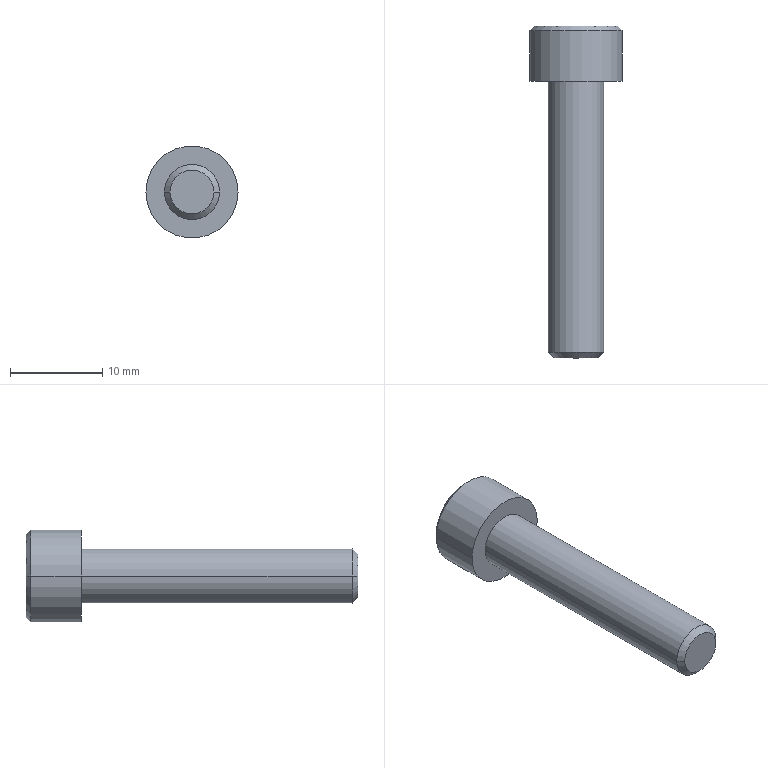Component | SolidWorks | TAD01-M6-L30Screw-2 | 1 solid | 25 faces | box 10 x 36 x 10 mm | volume 1238 mm3 | plane 15 | cone 6 | cylinder 4 | commonest cylinder face diameters 6 x2 10 x2
STEP:
#1=COLOUR_RGB('',0.7922,0.8196,0.9333);
#2=FILL_AREA_STYLE_COLOUR('',#1);
#3=FILL_AREA_STYLE('',(#2));
#4=SURFACE_STYLE_FILL_AREA(#3);
#5=SURFACE_SIDE_STYLE('',(#4));
#6=SURFACE_STYLE_USAGE(.BOTH.,#5);
#7=PRESENTATION_STYLE_ASSIGNMENT((#6));
#8=CARTESIAN_POINT('',(-0.1442,1.796,7.539));
#9=VERTEX_POINT('',#8);
#10=CARTESIAN_POINT('',(-0.3805,1.796,7.539));
#11=VERTEX_POINT('',#10);
#12=CARTESIAN_POINT('',(-0.2623,1.796,7.539));
#13=DIRECTION('',(0.,1.,0.));
#14=DIRECTION('',(1.,0.,0.));
#15=AXIS2_PLACEMENT_3D('',#12,#13,#14);
#16=CIRCLE('',#15,0.1181);
#17=EDGE_CURVE('',#9,#11,#16,.T.);
#18=ORIENTED_EDGE('',*,*,#17,.T.);
#19=CARTESIAN_POINT('',(-0.3805,2.953,7.539));
#20=VERTEX_POINT('',#19);
#21=CARTESIAN_POINT('',(-0.3805,1.771,7.539));
#22=DIRECTION('',(0.,1.,0.));
#23=VECTOR('',#22,39.37);
#24=LINE('',#21,#23);
#25=EDGE_CURVE('',#11,#20,#24,.T.);
#26=ORIENTED_EDGE('',*,*,#25,.T.);
#27=CARTESIAN_POINT('',(-0.1442,2.953,7.539));
#28=VERTEX_POINT('',#27);
#29=CARTESIAN_POINT('',(-0.2623,2.953,7.539));
#30=DIRECTION('',(0.,-1.,0.));
#31=DIRECTION('',(1.,0.,0.));
#32=AXIS2_PLACEMENT_3D('',#29,#30,#31);
#33=CIRCLE('',#32,0.1181);
#34=EDGE_CURVE('',#20,#28,#33,.T.);
#35=ORIENTED_EDGE('',*,*,#34,.T.);
#36=CARTESIAN_POINT('',(-0.1442,1.771,7.539));
#37=DIRECTION('',(0.,1.,0.));
#38=VECTOR('',#37,39.37);
#39=LINE('',#36,#38);
#40=EDGE_CURVE('',#9,#28,#39,.T.);
#41=ORIENTED_EDGE('',*,*,#40,.F.);
#42=EDGE_LOOP('',(#18,#26,#35,#41));
#43=FACE_OUTER_BOUND('',#42,.T.);
#44=CARTESIAN_POINT('',(-0.2623,1.771,7.539));
#45=DIRECTION('',(0.,1.,0.));
#46=DIRECTION('',(1.,0.,0.));
#47=AXIS2_PLACEMENT_3D('',#44,#45,#46);
#48=CYLINDRICAL_SURFACE('',#47,0.1181);
#49=ADVANCED_FACE('',(#43),#48,.T.);
#50=CARTESIAN_POINT('',(-0.1684,1.771,7.539));
#51=VERTEX_POINT('',#50);
#52=CARTESIAN_POINT('',(-0.3563,1.771,7.539));
#53=VERTEX_POINT('',#52);
#54=CARTESIAN_POINT('',(-0.2623,1.771,7.539));
#55=DIRECTION('',(0.,1.,0.));
#56=DIRECTION('',(1.,0.,0.));
#57=AXIS2_PLACEMENT_3D('',#54,#55,#56);
#58=CIRCLE('',#57,0.09396);
#59=EDGE_CURVE('',#51,#53,#58,.T.);
#60=ORIENTED_EDGE('',*,*,#59,.T.);
#61=CARTESIAN_POINT('',(-0.3805,1.796,7.539));
#62=DIRECTION('',(-0.7071,0.7071,-0.));
#63=VECTOR('',#62,39.37);
#64=LINE('',#61,#63);
#65=EDGE_CURVE('',#53,#11,#64,.T.);
#66=ORIENTED_EDGE('',*,*,#65,.T.);
#67=ORIENTED_EDGE('',*,*,#17,.F.);
#68=CARTESIAN_POINT('',(-0.1442,1.796,7.539));
#69=DIRECTION('',(0.7071,0.7071,0.));
#70=VECTOR('',#69,39.37);
#71=LINE('',#68,#70);
#72=EDGE_CURVE('',#51,#9,#71,.T.);
#73=ORIENTED_EDGE('',*,*,#72,.F.);
#74=EDGE_LOOP('',(#60,#66,#67,#73));
#75=FACE_OUTER_BOUND('',#74,.T.);
#76=CARTESIAN_POINT('',(-0.2623,1.796,7.539));
#77=DIRECTION('',(0.,1.,0.));
#78=DIRECTION('',(1.,0.,0.));
#79=AXIS2_PLACEMENT_3D('',#76,#77,#78);
#80=CONICAL_SURFACE('',#79,0.1181,0.7854);
#81=ADVANCED_FACE('',(#75),#80,.T.);
#82=CARTESIAN_POINT('',(-0.06549,2.953,7.539));
#83=VERTEX_POINT('',#82);
#84=CARTESIAN_POINT('',(-0.4592,2.953,7.539));
#85=VERTEX_POINT('',#84);
#86=CARTESIAN_POINT('',(-0.2623,2.953,7.539));
#87=DIRECTION('',(0.,1.,0.));
#88=DIRECTION('',(1.,0.,0.));
#89=AXIS2_PLACEMENT_3D('',#86,#87,#88);
#90=CIRCLE('',#89,0.1969);
#91=EDGE_CURVE('',#83,#85,#90,.T.);
#92=ORIENTED_EDGE('',*,*,#91,.T.);
#93=CARTESIAN_POINT('',(-0.4592,3.169,7.539));
#94=VERTEX_POINT('',#93);
#95=CARTESIAN_POINT('',(-0.4592,2.953,7.539));
#96=DIRECTION('',(0.,1.,0.));
#97=VECTOR('',#96,39.37);
#98=LINE('',#95,#97);
#99=EDGE_CURVE('',#85,#94,#98,.T.);
#100=ORIENTED_EDGE('',*,*,#99,.T.);
#101=CARTESIAN_POINT('',(-0.06549,3.169,7.539));
#102=VERTEX_POINT('',#101);
#103=CARTESIAN_POINT('',(-0.2623,3.169,7.539));
#104=DIRECTION('',(0.,-1.,0.));
#105=DIRECTION('',(1.,0.,0.));
#106=AXIS2_PLACEMENT_3D('',#103,#104,#105);
#107=CIRCLE('',#106,0.1969);
#108=EDGE_CURVE('',#94,#102,#107,.T.);
#109=ORIENTED_EDGE('',*,*,#108,.T.);
#110=CARTESIAN_POINT('',(-0.06549,2.953,7.539));
#111=DIRECTION('',(0.,1.,0.));
#112=VECTOR('',#111,39.37);
#113=LINE('',#110,#112);
#114=EDGE_CURVE('',#83,#102,#113,.T.);
#115=ORIENTED_EDGE('',*,*,#114,.F.);
#116=EDGE_LOOP('',(#92,#100,#109,#115));
#117=FACE_OUTER_BOUND('',#116,.T.);
#118=CARTESIAN_POINT('',(-0.2623,2.953,7.539));
#119=DIRECTION('',(0.,1.,0.));
#120=DIRECTION('',(1.,0.,0.));
#121=AXIS2_PLACEMENT_3D('',#118,#119,#120);
#122=CYLINDRICAL_SURFACE('',#121,0.1969);
#123=ADVANCED_FACE('',(#117),#122,.T.);
#124=CARTESIAN_POINT('',(-0.4395,3.189,7.539));
#125=VERTEX_POINT('',#124);
#126=CARTESIAN_POINT('',(-0.08518,3.189,7.539));
#127=VERTEX_POINT('',#126);
#128=CARTESIAN_POINT('',(-0.2623,3.189,7.539));
#129=DIRECTION('',(0.,-1.,0.));
#130=DIRECTION('',(-1.,0.,0.));
#131=AXIS2_PLACEMENT_3D('',#128,#129,#130);
#132=CIRCLE('',#131,0.1772);
#133=EDGE_CURVE('',#125,#127,#132,.T.);
#134=ORIENTED_EDGE('',*,*,#133,.T.);
#135=CARTESIAN_POINT('',(-0.06549,3.169,7.539));
#136=DIRECTION('',(0.7071,-0.7071,-0.));
#137=VECTOR('',#136,39.37);
#138=LINE('',#135,#137);
#139=EDGE_CURVE('',#127,#102,#138,.T.);
#140=ORIENTED_EDGE('',*,*,#139,.T.);
#141=ORIENTED_EDGE('',*,*,#108,.F.);
#142=CARTESIAN_POINT('',(-0.4592,3.169,7.539));
#143=DIRECTION('',(-0.7071,-0.7071,0.));
#144=VECTOR('',#143,39.37);
#145=LINE('',#142,#144);
#146=EDGE_CURVE('',#125,#94,#145,.T.);
#147=ORIENTED_EDGE('',*,*,#146,.F.);
#148=EDGE_LOOP('',(#134,#140,#141,#147));
#149=FACE_OUTER_BOUND('',#148,.T.);
#150=CARTESIAN_POINT('',(-0.2623,3.169,7.539));
#151=DIRECTION('',(0.,-1.,0.));
#152=DIRECTION('',(-1.,0.,0.));
#153=AXIS2_PLACEMENT_3D('',#150,#151,#152);
#154=CONICAL_SURFACE('',#153,0.1969,0.7854);
#155=ADVANCED_FACE('',(#149),#154,.T.);
#156=CARTESIAN_POINT('',(-0.2623,3.014,7.539));
#157=VERTEX_POINT('',#156);
#158=CARTESIAN_POINT('',(-0.2623,3.071,7.638));
#159=VERTEX_POINT('',#158);
#160=CARTESIAN_POINT('',(-0.2623,3.071,7.638));
#161=DIRECTION('',(0.,0.5,0.866));
#162=VECTOR('',#161,39.37);
#163=LINE('',#160,#162);
#164=EDGE_CURVE('',#157,#159,#163,.T.);
#165=ORIENTED_EDGE('',*,*,#164,.F.);
#166=CARTESIAN_POINT('',(-0.2623,3.071,7.441));
#167=VERTEX_POINT('',#166);
#168=CARTESIAN_POINT('',(-0.2623,3.071,7.441));
#169=DIRECTION('',(0.,0.5,-0.866));
#170=VECTOR('',#169,39.37);
#171=LINE('',#168,#170);
#172=EDGE_CURVE('',#157,#167,#171,.T.);
#173=ORIENTED_EDGE('',*,*,#172,.T.);
#174=CARTESIAN_POINT('',(-0.3116,3.071,7.454));
#175=VERTEX_POINT('',#174);
#176=CARTESIAN_POINT('',(-0.2623,3.071,7.539));
#177=DIRECTION('',(-0.,-1.,-0.));
#178=DIRECTION('',(0.,0.,1.));
#179=AXIS2_PLACEMENT_3D('',#176,#177,#178);
#180=CIRCLE('',#179,0.09843);
#181=EDGE_CURVE('',#175,#167,#180,.T.);
#182=ORIENTED_EDGE('',*,*,#181,.F.);
#183=CARTESIAN_POINT('',(-0.3608,3.071,7.539));
#184=VERTEX_POINT('',#183);
#185=CARTESIAN_POINT('',(-0.2623,3.071,7.539));
#186=DIRECTION('',(-0.,-1.,-0.));
#187=DIRECTION('',(-0.,0.,1.));
#188=AXIS2_PLACEMENT_3D('',#185,#186,#187);
#189=CIRCLE('',#188,0.09843);
#190=EDGE_CURVE('',#184,#175,#189,.T.);
#191=ORIENTED_EDGE('',*,*,#190,.F.);
#192=CARTESIAN_POINT('',(-0.3116,3.071,7.625));
#193=VERTEX_POINT('',#192);
#194=CARTESIAN_POINT('',(-0.2623,3.071,7.539));
#195=DIRECTION('',(-0.,-1.,-0.));
#196=DIRECTION('',(0.,0.,1.));
#197=AXIS2_PLACEMENT_3D('',#194,#195,#196);
#198=CIRCLE('',#197,0.09843);
#199=EDGE_CURVE('',#193,#184,#198,.T.);
#200=ORIENTED_EDGE('',*,*,#199,.F.);
#201=CARTESIAN_POINT('',(-0.2623,3.071,7.539));
#202=DIRECTION('',(-0.,-1.,-0.));
#203=DIRECTION('',(0.,0.,1.));
#204=AXIS2_PLACEMENT_3D('',#201,#202,#203);
#205=CIRCLE('',#204,0.09843);
#206=EDGE_CURVE('',#159,#193,#205,.T.);
#207=ORIENTED_EDGE('',*,*,#206,.F.);
#208=EDGE_LOOP('',(#165,#173,#182,#191,#200,#207));
#209=FACE_OUTER_BOUND('',#208,.T.);
#210=CARTESIAN_POINT('',(-0.2623,3.071,7.539));
#211=DIRECTION('',(0.,1.,0.));
#212=DIRECTION('',(0.,0.,1.));
#213=AXIS2_PLACEMENT_3D('',#210,#211,#212);
#214=CONICAL_SURFACE('',#213,0.09843,1.047);
#215=ADVANCED_FACE('',(#209),#214,.F.);
#216=ORIENTED_EDGE('',*,*,#25,.F.);
#217=CARTESIAN_POINT('',(-0.2623,1.796,7.539));
#218=DIRECTION('',(0.,1.,0.));
#219=DIRECTION('',(1.,0.,0.));
#220=AXIS2_PLACEMENT_3D('',#217,#218,#219);
#221=CIRCLE('',#220,0.1181);
#222=EDGE_CURVE('',#11,#9,#221,.T.);
#223=ORIENTED_EDGE('',*,*,#222,.T.);
#224=ORIENTED_EDGE('',*,*,#40,.T.);
#225=CARTESIAN_POINT('',(-0.2623,2.953,7.539));
#226=DIRECTION('',(0.,-1.,0.));
#227=DIRECTION('',(1.,0.,0.));
#228=AXIS2_PLACEMENT_3D('',#225,#226,#227);
#229=CIRCLE('',#228,0.1181);
#230=EDGE_CURVE('',#28,#20,#229,.T.);
#231=ORIENTED_EDGE('',*,*,#230,.T.);
#232=EDGE_LOOP('',(#216,#223,#224,#231));
#233=FACE_OUTER_BOUND('',#232,.T.);
#234=CARTESIAN_POINT('',(-0.2623,1.771,7.539));
#235=DIRECTION('',(0.,1.,0.));
#236=DIRECTION('',(1.,0.,0.));
#237=AXIS2_PLACEMENT_3D('',#234,#235,#236);
#238=CYLINDRICAL_SURFACE('',#237,0.1181);
#239=ADVANCED_FACE('',(#233),#238,.T.);
#240=ORIENTED_EDGE('',*,*,#91,.F.);
#241=CARTESIAN_POINT('',(-0.2623,2.953,7.539));
#242=DIRECTION('',(0.,1.,0.));
#243=DIRECTION('',(1.,0.,0.));
#244=AXIS2_PLACEMENT_3D('',#241,#242,#243);
#245=CIRCLE('',#244,0.1969);
#246=EDGE_CURVE('',#85,#83,#245,.T.);
#247=ORIENTED_EDGE('',*,*,#246,.F.);
#248=EDGE_LOOP('',(#240,#247));
#249=FACE_OUTER_BOUND('',#248,.T.);
#250=ORIENTED_EDGE('',*,*,#230,.F.);
#251=ORIENTED_EDGE('',*,*,#34,.F.);
#252=EDGE_LOOP('',(#250,#251));
#253=FACE_BOUND('',#252,.T.);
#254=CARTESIAN_POINT('',(-0.2623,2.953,7.343));
#255=DIRECTION('',(0.,1.,0.));
#256=DIRECTION('',(1.,0.,0.));
#257=AXIS2_PLACEMENT_3D('',#254,#255,#256);
#258=PLANE('',#257);
#259=ADVANCED_FACE('',(#249,#253),#258,.F.);
#260=ORIENTED_EDGE('',*,*,#65,.F.);
#261=CARTESIAN_POINT('',(-0.2623,1.771,7.539));
#262=DIRECTION('',(0.,1.,0.));
#263=DIRECTION('',(1.,0.,0.));
#264=AXIS2_PLACEMENT_3D('',#261,#262,#263);
#265=CIRCLE('',#264,0.09396);
#266=EDGE_CURVE('',#53,#51,#265,.T.);
#267=ORIENTED_EDGE('',*,*,#266,.T.);
#268=ORIENTED_EDGE('',*,*,#72,.T.);
#269=ORIENTED_EDGE('',*,*,#222,.F.);
#270=EDGE_LOOP('',(#260,#267,#268,#269));
#271=FACE_OUTER_BOUND('',#270,.T.);
#272=CARTESIAN_POINT('',(-0.2623,1.796,7.539));
#273=DIRECTION('',(0.,1.,0.));
#274=DIRECTION('',(1.,0.,0.));
#275=AXIS2_PLACEMENT_3D('',#272,#273,#274);
#276=CONICAL_SURFACE('',#275,0.1181,0.7854);
#277=ADVANCED_FACE('',(#271),#276,.T.);
#278=ORIENTED_EDGE('',*,*,#99,.F.);
#279=ORIENTED_EDGE('',*,*,#246,.T.);
#280=ORIENTED_EDGE('',*,*,#114,.T.);
#281=CARTESIAN_POINT('',(-0.2623,3.169,7.539));
#282=DIRECTION('',(0.,-1.,0.));
#283=DIRECTION('',(1.,0.,0.));
#284=AXIS2_PLACEMENT_3D('',#281,#282,#283);
#285=CIRCLE('',#284,0.1969);
#286=EDGE_CURVE('',#102,#94,#285,.T.);
#287=ORIENTED_EDGE('',*,*,#286,.T.);
#288=EDGE_LOOP('',(#278,#279,#280,#287));
#289=FACE_OUTER_BOUND('',#288,.T.);
#290=CARTESIAN_POINT('',(-0.2623,2.953,7.539));
#291=DIRECTION('',(0.,1.,0.));
#292=DIRECTION('',(1.,0.,0.));
#293=AXIS2_PLACEMENT_3D('',#290,#291,#292);
#294=CYLINDRICAL_SURFACE('',#293,0.1969);
#295=ADVANCED_FACE('',(#289),#294,.T.);
#296=ORIENTED_EDGE('',*,*,#59,.F.);
#297=ORIENTED_EDGE('',*,*,#266,.F.);
#298=EDGE_LOOP('',(#296,#297));
#299=FACE_OUTER_BOUND('',#298,.T.);
#300=CARTESIAN_POINT('',(-0.2623,1.771,7.445));
#301=DIRECTION('',(0.,1.,0.));
#302=DIRECTION('',(1.,0.,0.));
#303=AXIS2_PLACEMENT_3D('',#300,#301,#302);
#304=PLANE('',#303);
#305=ADVANCED_FACE('',(#299),#304,.F.);
#306=ORIENTED_EDGE('',*,*,#139,.F.);
#307=CARTESIAN_POINT('',(-0.2623,3.189,7.539));
#308=DIRECTION('',(0.,-1.,0.));
#309=DIRECTION('',(-1.,0.,0.));
#310=AXIS2_PLACEMENT_3D('',#307,#308,#309);
#311=CIRCLE('',#310,0.1772);
#312=EDGE_CURVE('',#127,#125,#311,.T.);
#313=ORIENTED_EDGE('',*,*,#312,.T.);
#314=ORIENTED_EDGE('',*,*,#146,.T.);
#315=ORIENTED_EDGE('',*,*,#286,.F.);
#316=EDGE_LOOP('',(#306,#313,#314,#315));
#317=FACE_OUTER_BOUND('',#316,.T.);
#318=CARTESIAN_POINT('',(-0.2623,3.169,7.539));
#319=DIRECTION('',(0.,-1.,0.));
#320=DIRECTION('',(-1.,0.,0.));
#321=AXIS2_PLACEMENT_3D('',#318,#319,#320);
#322=CONICAL_SURFACE('',#321,0.1969,0.7854);
#323=ADVANCED_FACE('',(#317),#322,.T.);
#324=CARTESIAN_POINT('',(-0.3608,3.189,7.596));
#325=VERTEX_POINT('',#324);
#326=CARTESIAN_POINT('',(-0.2623,3.189,7.653));
#327=VERTEX_POINT('',#326);
#328=CARTESIAN_POINT('',(-0.3608,3.189,7.596));
#329=DIRECTION('',(0.866,0.,0.5));
#330=VECTOR('',#329,39.37);
#331=LINE('',#328,#330);
#332=EDGE_CURVE('',#325,#327,#331,.T.);
#333=ORIENTED_EDGE('',*,*,#332,.F.);
#334=CARTESIAN_POINT('',(-0.3608,3.189,7.483));
#335=VERTEX_POINT('',#334);
#336=CARTESIAN_POINT('',(-0.3608,3.189,7.539));
#337=DIRECTION('',(0.,0.,1.));
#338=VECTOR('',#337,39.37);
#339=LINE('',#336,#338);
#340=EDGE_CURVE('',#335,#325,#339,.T.);
#341=ORIENTED_EDGE('',*,*,#340,.F.);
#342=CARTESIAN_POINT('',(-0.2623,3.189,7.426));
#343=VERTEX_POINT('',#342);
#344=CARTESIAN_POINT('',(-0.2623,3.189,7.426));
#345=DIRECTION('',(-0.866,0.,0.5));
#346=VECTOR('',#345,39.37);
#347=LINE('',#344,#346);
#348=EDGE_CURVE('',#343,#335,#347,.T.);
#349=ORIENTED_EDGE('',*,*,#348,.F.);
#350=CARTESIAN_POINT('',(-0.1639,3.189,7.483));
#351=VERTEX_POINT('',#350);
#352=CARTESIAN_POINT('',(-0.1639,3.189,7.483));
#353=DIRECTION('',(-0.866,0.,-0.5));
#354=VECTOR('',#353,39.37);
#355=LINE('',#352,#354);
#356=EDGE_CURVE('',#351,#343,#355,.T.);
#357=ORIENTED_EDGE('',*,*,#356,.F.);
#358=CARTESIAN_POINT('',(-0.1639,3.189,7.596));
#359=VERTEX_POINT('',#358);
#360=CARTESIAN_POINT('',(-0.1639,3.189,7.539));
#361=DIRECTION('',(0.,0.,-1.));
#362=VECTOR('',#361,39.37);
#363=LINE('',#360,#362);
#364=EDGE_CURVE('',#359,#351,#363,.T.);
#365=ORIENTED_EDGE('',*,*,#364,.F.);
#366=CARTESIAN_POINT('',(-0.2623,3.189,7.653));
#367=DIRECTION('',(0.866,0.,-0.5));
#368=VECTOR('',#367,39.37);
#369=LINE('',#366,#368);
#370=EDGE_CURVE('',#327,#359,#369,.T.);
#371=ORIENTED_EDGE('',*,*,#370,.F.);
#372=EDGE_LOOP('',(#333,#341,#349,#357,#365,#371));
#373=FACE_BOUND('',#372,.T.);
#374=ORIENTED_EDGE('',*,*,#133,.F.);
#375=ORIENTED_EDGE('',*,*,#312,.F.);
#376=EDGE_LOOP('',(#374,#375));
#377=FACE_OUTER_BOUND('',#376,.T.);
#378=CARTESIAN_POINT('',(-0.2623,3.189,7.539));
#379=DIRECTION('',(0.,-1.,0.));
#380=DIRECTION('',(-1.,0.,0.));
#381=AXIS2_PLACEMENT_3D('',#378,#379,#380);
#382=PLANE('',#381);
#383=ADVANCED_FACE('',(#373,#377),#382,.F.);
#384=CARTESIAN_POINT('',(-0.1639,3.071,7.596));
#385=VERTEX_POINT('',#384);
#386=CARTESIAN_POINT('',(-0.1639,3.071,7.596));
#387=DIRECTION('',(0.,1.,0.));
#388=VECTOR('',#387,39.37);
#389=LINE('',#386,#388);
#390=EDGE_CURVE('',#385,#359,#389,.T.);
#391=ORIENTED_EDGE('',*,*,#390,.F.);
#392=CARTESIAN_POINT('',(-0.2131,3.071,7.625));
#393=VERTEX_POINT('',#392);
#394=CARTESIAN_POINT('',(-0.2131,3.071,7.625));
#395=DIRECTION('',(0.866,0.,-0.5));
#396=VECTOR('',#395,39.37);
#397=LINE('',#394,#396);
#398=EDGE_CURVE('',#393,#385,#397,.T.);
#399=ORIENTED_EDGE('',*,*,#398,.F.);
#400=CARTESIAN_POINT('',(-0.2623,3.071,7.653));
#401=VERTEX_POINT('',#400);
#402=CARTESIAN_POINT('',(-0.2623,3.071,7.653));
#403=DIRECTION('',(0.866,0.,-0.5));
#404=VECTOR('',#403,39.37);
#405=LINE('',#402,#404);
#406=EDGE_CURVE('',#401,#393,#405,.T.);
#407=ORIENTED_EDGE('',*,*,#406,.F.);
#408=CARTESIAN_POINT('',(-0.2623,3.071,7.653));
#409=DIRECTION('',(0.,-1.,0.));
#410=VECTOR('',#409,39.37);
#411=LINE('',#408,#410);
#412=EDGE_CURVE('',#327,#401,#411,.T.);
#413=ORIENTED_EDGE('',*,*,#412,.F.);
#414=ORIENTED_EDGE('',*,*,#370,.T.);
#415=EDGE_LOOP('',(#391,#399,#407,#413,#414));
#416=FACE_OUTER_BOUND('',#415,.T.);
#417=CARTESIAN_POINT('',(-0.2623,3.071,7.653));
#418=DIRECTION('',(0.5,0.,0.866));
#419=DIRECTION('',(0.866,0.,-0.5));
#420=AXIS2_PLACEMENT_3D('',#417,#418,#419);
#421=PLANE('',#420);
#422=ADVANCED_FACE('',(#416),#421,.F.);
#423=ORIENTED_EDGE('',*,*,#412,.T.);
#424=CARTESIAN_POINT('',(-0.3116,3.071,7.625));
#425=DIRECTION('',(0.866,0.,0.5));
#426=VECTOR('',#425,39.37);
#427=LINE('',#424,#426);
#428=EDGE_CURVE('',#193,#401,#427,.T.);
#429=ORIENTED_EDGE('',*,*,#428,.F.);
#430=CARTESIAN_POINT('',(-0.3608,3.071,7.596));
#431=VERTEX_POINT('',#430);
#432=CARTESIAN_POINT('',(-0.3608,3.071,7.596));
#433=DIRECTION('',(0.866,0.,0.5));
#434=VECTOR('',#433,39.37);
#435=LINE('',#432,#434);
#436=EDGE_CURVE('',#431,#193,#435,.T.);
#437=ORIENTED_EDGE('',*,*,#436,.F.);
#438=CARTESIAN_POINT('',(-0.3608,3.071,7.596));
#439=DIRECTION('',(0.,-1.,0.));
#440=VECTOR('',#439,39.37);
#441=LINE('',#438,#440);
#442=EDGE_CURVE('',#325,#431,#441,.T.);
#443=ORIENTED_EDGE('',*,*,#442,.F.);
#444=ORIENTED_EDGE('',*,*,#332,.T.);
#445=EDGE_LOOP('',(#423,#429,#437,#443,#444));
#446=FACE_OUTER_BOUND('',#445,.T.);
#447=CARTESIAN_POINT('',(-0.3608,3.071,7.596));
#448=DIRECTION('',(-0.5,0.,0.866));
#449=DIRECTION('',(0.866,0.,0.5));
#450=AXIS2_PLACEMENT_3D('',#447,#448,#449);
#451=PLANE('',#450);
#452=ADVANCED_FACE('',(#446),#451,.F.);
#453=ORIENTED_EDGE('',*,*,#442,.T.);
#454=CARTESIAN_POINT('',(-0.3608,3.071,7.539));
#455=DIRECTION('',(0.,0.,1.));
#456=VECTOR('',#455,39.37);
#457=LINE('',#454,#456);
#458=EDGE_CURVE('',#184,#431,#457,.T.);
#459=ORIENTED_EDGE('',*,*,#458,.F.);
#460=CARTESIAN_POINT('',(-0.3608,3.071,7.483));
#461=VERTEX_POINT('',#460);
#462=CARTESIAN_POINT('',(-0.3608,3.071,7.539));
#463=DIRECTION('',(0.,0.,1.));
#464=VECTOR('',#463,39.37);
#465=LINE('',#462,#464);
#466=EDGE_CURVE('',#461,#184,#465,.T.);
#467=ORIENTED_EDGE('',*,*,#466,.F.);
#468=CARTESIAN_POINT('',(-0.3608,3.071,7.483));
#469=DIRECTION('',(0.,-1.,0.));
#470=VECTOR('',#469,39.37);
#471=LINE('',#468,#470);
#472=EDGE_CURVE('',#335,#461,#471,.T.);
#473=ORIENTED_EDGE('',*,*,#472,.F.);
#474=ORIENTED_EDGE('',*,*,#340,.T.);
#475=EDGE_LOOP('',(#453,#459,#467,#473,#474));
#476=FACE_OUTER_BOUND('',#475,.T.);
#477=CARTESIAN_POINT('',(-0.3608,3.071,7.483));
#478=DIRECTION('',(-1.,0.,0.));
#479=DIRECTION('',(0.,1.,0.));
#480=AXIS2_PLACEMENT_3D('',#477,#478,#479);
#481=PLANE('',#480);
#482=ADVANCED_FACE('',(#476),#481,.F.);
#483=ORIENTED_EDGE('',*,*,#472,.T.);
#484=CARTESIAN_POINT('',(-0.3116,3.071,7.454));
#485=DIRECTION('',(-0.866,0.,0.5));
#486=VECTOR('',#485,39.37);
#487=LINE('',#484,#486);
#488=EDGE_CURVE('',#175,#461,#487,.T.);
#489=ORIENTED_EDGE('',*,*,#488,.F.);
#490=CARTESIAN_POINT('',(-0.2623,3.071,7.426));
#491=VERTEX_POINT('',#490);
#492=CARTESIAN_POINT('',(-0.2623,3.071,7.426));
#493=DIRECTION('',(-0.866,0.,0.5));
#494=VECTOR('',#493,39.37);
#495=LINE('',#492,#494);
#496=EDGE_CURVE('',#491,#175,#495,.T.);
#497=ORIENTED_EDGE('',*,*,#496,.F.);
#498=CARTESIAN_POINT('',(-0.2623,3.071,7.426));
#499=DIRECTION('',(0.,-1.,0.));
#500=VECTOR('',#499,39.37);
#501=LINE('',#498,#500);
#502=EDGE_CURVE('',#343,#491,#501,.T.);
#503=ORIENTED_EDGE('',*,*,#502,.F.);
#504=ORIENTED_EDGE('',*,*,#348,.T.);
#505=EDGE_LOOP('',(#483,#489,#497,#503,#504));
#506=FACE_OUTER_BOUND('',#505,.T.);
#507=CARTESIAN_POINT('',(-0.2623,3.071,7.426));
#508=DIRECTION('',(-0.5,0.,-0.866));
#509=DIRECTION('',(-0.866,0.,0.5));
#510=AXIS2_PLACEMENT_3D('',#507,#508,#509);
#511=PLANE('',#510);
#512=ADVANCED_FACE('',(#506),#511,.F.);
#513=ORIENTED_EDGE('',*,*,#502,.T.);
#514=CARTESIAN_POINT('',(-0.2131,3.071,7.454));
#515=VERTEX_POINT('',#514);
#516=CARTESIAN_POINT('',(-0.2131,3.071,7.454));
#517=DIRECTION('',(-0.866,0.,-0.5));
#518=VECTOR('',#517,39.37);
#519=LINE('',#516,#518);
#520=EDGE_CURVE('',#515,#491,#519,.T.);
#521=ORIENTED_EDGE('',*,*,#520,.F.);
#522=CARTESIAN_POINT('',(-0.1639,3.071,7.483));
#523=VERTEX_POINT('',#522);
#524=CARTESIAN_POINT('',(-0.1639,3.071,7.483));
#525=DIRECTION('',(-0.866,0.,-0.5));
#526=VECTOR('',#525,39.37);
#527=LINE('',#524,#526);
#528=EDGE_CURVE('',#523,#515,#527,.T.);
#529=ORIENTED_EDGE('',*,*,#528,.F.);
#530=CARTESIAN_POINT('',(-0.1639,3.071,7.483));
#531=DIRECTION('',(0.,-1.,0.));
#532=VECTOR('',#531,39.37);
#533=LINE('',#530,#532);
#534=EDGE_CURVE('',#351,#523,#533,.T.);
#535=ORIENTED_EDGE('',*,*,#534,.F.);
#536=ORIENTED_EDGE('',*,*,#356,.T.);
#537=EDGE_LOOP('',(#513,#521,#529,#535,#536));
#538=FACE_OUTER_BOUND('',#537,.T.);
#539=CARTESIAN_POINT('',(-0.1639,3.071,7.483));
#540=DIRECTION('',(0.5,0.,-0.866));
#541=DIRECTION('',(-0.866,0.,-0.5));
#542=AXIS2_PLACEMENT_3D('',#539,#540,#541);
#543=PLANE('',#542);
#544=ADVANCED_FACE('',(#538),#543,.F.);
#545=ORIENTED_EDGE('',*,*,#534,.T.);
#546=CARTESIAN_POINT('',(-0.1639,3.071,7.539));
#547=VERTEX_POINT('',#546);
#548=CARTESIAN_POINT('',(-0.1639,3.071,7.596));
#549=DIRECTION('',(0.,0.,-1.));
#550=VECTOR('',#549,39.37);
#551=LINE('',#548,#550);
#552=EDGE_CURVE('',#547,#523,#551,.T.);
#553=ORIENTED_EDGE('',*,*,#552,.F.);
#554=CARTESIAN_POINT('',(-0.1639,3.071,7.539));
#555=DIRECTION('',(0.,0.,-1.));
#556=VECTOR('',#555,39.37);
#557=LINE('',#554,#556);
#558=EDGE_CURVE('',#385,#547,#557,.T.);
#559=ORIENTED_EDGE('',*,*,#558,.F.);
#560=ORIENTED_EDGE('',*,*,#390,.T.);
#561=ORIENTED_EDGE('',*,*,#364,.T.);
#562=EDGE_LOOP('',(#545,#553,#559,#560,#561));
#563=FACE_OUTER_BOUND('',#562,.T.);
#564=CARTESIAN_POINT('',(-0.1639,3.071,7.596));
#565=DIRECTION('',(1.,0.,0.));
#566=DIRECTION('',(0.,-1.,0.));
#567=AXIS2_PLACEMENT_3D('',#564,#565,#566);
#568=PLANE('',#567);
#569=ADVANCED_FACE('',(#563),#568,.F.);
#570=CARTESIAN_POINT('',(-0.2623,3.071,7.539));
#571=DIRECTION('',(-0.,-1.,-0.));
#572=DIRECTION('',(0.,0.,1.));
#573=AXIS2_PLACEMENT_3D('',#570,#571,#572);
#574=CIRCLE('',#573,0.09843);
#575=EDGE_CURVE('',#515,#547,#574,.T.);
#576=ORIENTED_EDGE('',*,*,#575,.T.);
#577=ORIENTED_EDGE('',*,*,#552,.T.);
#578=ORIENTED_EDGE('',*,*,#528,.T.);
#579=EDGE_LOOP('',(#576,#577,#578));
#580=FACE_OUTER_BOUND('',#579,.T.);
#581=CARTESIAN_POINT('',(-0.2623,3.071,7.539));
#582=DIRECTION('',(0.,1.,0.));
#583=DIRECTION('',(1.,0.,0.));
#584=AXIS2_PLACEMENT_3D('',#581,#582,#583);
#585=PLANE('',#584);
#586=ADVANCED_FACE('',(#580),#585,.T.);
#587=ORIENTED_EDGE('',*,*,#172,.F.);
#588=ORIENTED_EDGE('',*,*,#164,.T.);
#589=CARTESIAN_POINT('',(-0.2623,3.071,7.539));
#590=DIRECTION('',(-0.,-1.,-0.));
#591=DIRECTION('',(0.,0.,1.));
#592=AXIS2_PLACEMENT_3D('',#589,#590,#591);
#593=CIRCLE('',#592,0.09843);
#594=EDGE_CURVE('',#393,#159,#593,.T.);
#595=ORIENTED_EDGE('',*,*,#594,.F.);
#596=CARTESIAN_POINT('',(-0.2623,3.071,7.539));
#597=DIRECTION('',(-0.,-1.,-0.));
#598=DIRECTION('',(-0.,0.,1.));
#599=AXIS2_PLACEMENT_3D('',#596,#597,#598);
#600=CIRCLE('',#599,0.09843);
#601=EDGE_CURVE('',#547,#393,#600,.T.);
#602=ORIENTED_EDGE('',*,*,#601,.F.);
#603=ORIENTED_EDGE('',*,*,#575,.F.);
#604=CARTESIAN_POINT('',(-0.2623,3.071,7.539));
#605=DIRECTION('',(-0.,-1.,-0.));
#606=DIRECTION('',(0.,0.,1.));
#607=AXIS2_PLACEMENT_3D('',#604,#605,#606);
#608=CIRCLE('',#607,0.09843);
#609=EDGE_CURVE('',#167,#515,#608,.T.);
#610=ORIENTED_EDGE('',*,*,#609,.F.);
#611=EDGE_LOOP('',(#587,#588,#595,#602,#603,#610));
#612=FACE_OUTER_BOUND('',#611,.T.);
#613=CARTESIAN_POINT('',(-0.2623,3.071,7.539));
#614=DIRECTION('',(0.,1.,0.));
#615=DIRECTION('',(0.,0.,1.));
#616=AXIS2_PLACEMENT_3D('',#613,#614,#615);
#617=CONICAL_SURFACE('',#616,0.09843,1.047);
#618=ADVANCED_FACE('',(#612),#617,.F.);
#619=ORIENTED_EDGE('',*,*,#181,.T.);
#620=ORIENTED_EDGE('',*,*,#609,.T.);
#621=ORIENTED_EDGE('',*,*,#520,.T.);
#622=ORIENTED_EDGE('',*,*,#496,.T.);
#623=EDGE_LOOP('',(#619,#620,#621,#622));
#624=FACE_OUTER_BOUND('',#623,.T.);
#625=CARTESIAN_POINT('',(-0.2623,3.071,7.539));
#626=DIRECTION('',(0.,1.,0.));
#627=DIRECTION('',(1.,0.,0.));
#628=AXIS2_PLACEMENT_3D('',#625,#626,#627);
#629=PLANE('',#628);
#630=ADVANCED_FACE('',(#624),#629,.T.);
#631=ORIENTED_EDGE('',*,*,#190,.T.);
#632=ORIENTED_EDGE('',*,*,#488,.T.);
#633=ORIENTED_EDGE('',*,*,#466,.T.);
#634=EDGE_LOOP('',(#631,#632,#633));
#635=FACE_OUTER_BOUND('',#634,.T.);
#636=CARTESIAN_POINT('',(-0.2623,3.071,7.539));
#637=DIRECTION('',(0.,1.,0.));
#638=DIRECTION('',(1.,0.,0.));
#639=AXIS2_PLACEMENT_3D('',#636,#637,#638);
#640=PLANE('',#639);
#641=ADVANCED_FACE('',(#635),#640,.T.);
#642=ORIENTED_EDGE('',*,*,#199,.T.);
#643=ORIENTED_EDGE('',*,*,#458,.T.);
#644=ORIENTED_EDGE('',*,*,#436,.T.);
#645=EDGE_LOOP('',(#642,#643,#644));
#646=FACE_OUTER_BOUND('',#645,.T.);
#647=CARTESIAN_POINT('',(-0.2623,3.071,7.539));
#648=DIRECTION('',(0.,1.,0.));
#649=DIRECTION('',(1.,0.,0.));
#650=AXIS2_PLACEMENT_3D('',#647,#648,#649);
#651=PLANE('',#650);
#652=ADVANCED_FACE('',(#646),#651,.T.);
#653=ORIENTED_EDGE('',*,*,#594,.T.);
#654=ORIENTED_EDGE('',*,*,#206,.T.);
#655=ORIENTED_EDGE('',*,*,#428,.T.);
#656=ORIENTED_EDGE('',*,*,#406,.T.);
#657=EDGE_LOOP('',(#653,#654,#655,#656));
#658=FACE_OUTER_BOUND('',#657,.T.);
#659=CARTESIAN_POINT('',(-0.2623,3.071,7.539));
#660=DIRECTION('',(0.,1.,0.));
#661=DIRECTION('',(1.,0.,0.));
#662=AXIS2_PLACEMENT_3D('',#659,#660,#661);
#663=PLANE('',#662);
#664=ADVANCED_FACE('',(#658),#663,.T.);
#665=ORIENTED_EDGE('',*,*,#601,.T.);
#666=ORIENTED_EDGE('',*,*,#398,.T.);
#667=ORIENTED_EDGE('',*,*,#558,.T.);
#668=EDGE_LOOP('',(#665,#666,#667));
#669=FACE_OUTER_BOUND('',#668,.T.);
#670=CARTESIAN_POINT('',(-0.2623,3.071,7.539));
#671=DIRECTION('',(0.,1.,0.));
#672=DIRECTION('',(1.,0.,0.));
#673=AXIS2_PLACEMENT_3D('',#670,#671,#672);
#674=PLANE('',#673);
#675=ADVANCED_FACE('',(#669),#674,.T.);
#676=CLOSED_SHELL('',(#49,#81,#123,#155,#215,#239,#259,#277,#295,#305,#323,#383,#422,#452,#482,#512,#544,#569,#586,#618,#630,#641,#652,#664,#675));
#677=MANIFOLD_SOLID_BREP('',#676);
#678=STYLED_ITEM('',(#7),#677);
#679=PRESENTATION_LAYER_ASSIGNMENT('','',(#678));
#680=(LENGTH_UNIT()NAMED_UNIT(*)SI_UNIT($,.METRE.));
#681=LENGTH_MEASURE_WITH_UNIT(LENGTH_MEASURE(0.0254),#680);
#682=DIMENSIONAL_EXPONENTS(1.,0.,0.,0.,0.,0.,0.);
#683=(CONVERSION_BASED_UNIT('',#681)LENGTH_UNIT()NAMED_UNIT(#682));
#684=UNCERTAINTY_MEASURE_WITH_UNIT(LENGTH_MEASURE(0.00001),#683,'','');
#685=(NAMED_UNIT(*)PLANE_ANGLE_UNIT()SI_UNIT($,.RADIAN.));
#686=(NAMED_UNIT(*)SI_UNIT($,.STERADIAN.)SOLID_ANGLE_UNIT());
#687=(GEOMETRIC_REPRESENTATION_CONTEXT(3)GLOBAL_UNCERTAINTY_ASSIGNED_CONTEXT((#684))GLOBAL_UNIT_ASSIGNED_CONTEXT((#683,#685,#686))REPRESENTATION_CONTEXT('',''));
#688=MECHANICAL_DESIGN_GEOMETRIC_PRESENTATION_REPRESENTATION('',(#678),#687);
#689=CARTESIAN_POINT('',(0.,0.,0.));
#690=DIRECTION('',(0.,0.,1.));
#691=DIRECTION('',(1.,0.,0.));
#692=AXIS2_PLACEMENT_3D('',#689,#690,#691);
#693=(LENGTH_UNIT()NAMED_UNIT(*)SI_UNIT($,.METRE.));
#694=LENGTH_MEASURE_WITH_UNIT(LENGTH_MEASURE(0.0254),#693);
#695=DIMENSIONAL_EXPONENTS(1.,0.,0.,0.,0.,0.,0.);
#696=(CONVERSION_BASED_UNIT('',#694)LENGTH_UNIT()NAMED_UNIT(#695));
#697=UNCERTAINTY_MEASURE_WITH_UNIT(LENGTH_MEASURE(0.00001),#696,'','');
#698=(NAMED_UNIT(*)PLANE_ANGLE_UNIT()SI_UNIT($,.RADIAN.));
#699=(NAMED_UNIT(*)SI_UNIT($,.STERADIAN.)SOLID_ANGLE_UNIT());
#700=(GEOMETRIC_REPRESENTATION_CONTEXT(3)GLOBAL_UNCERTAINTY_ASSIGNED_CONTEXT((#697))GLOBAL_UNIT_ASSIGNED_CONTEXT((#696,#698,#699))REPRESENTATION_CONTEXT('',''));
#701=ADVANCED_BREP_SHAPE_REPRESENTATION('',(#677,#692),#700);